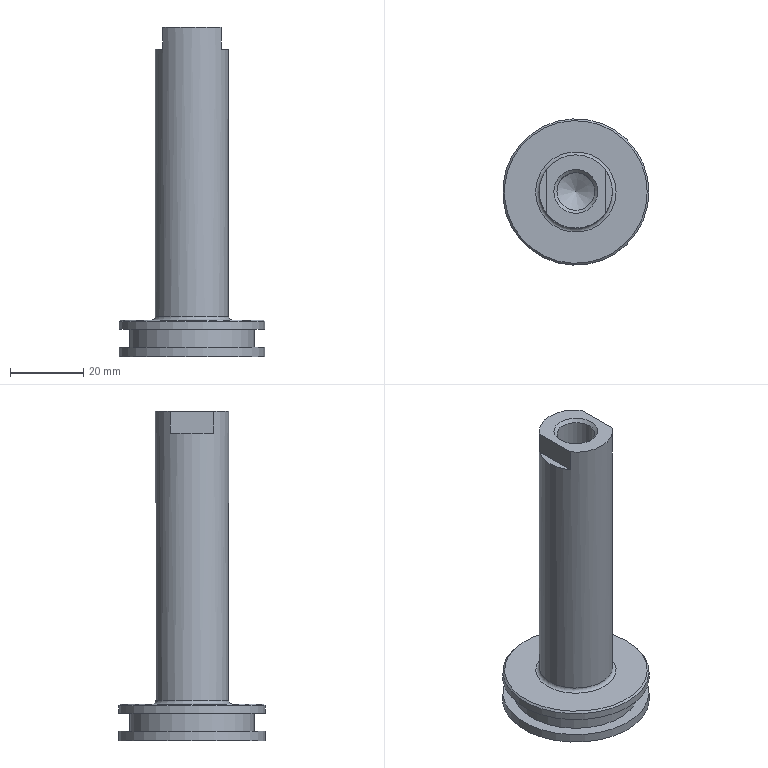Component | NX | PISTON_ROD | 1 solid | 18 faces | volume 34159 mm3 | plane 9 | cylinder 5 | cone 3 | torus 1 | commonest cylinder face diameters 40 x2 20 x1 34 x1 10.3 x1